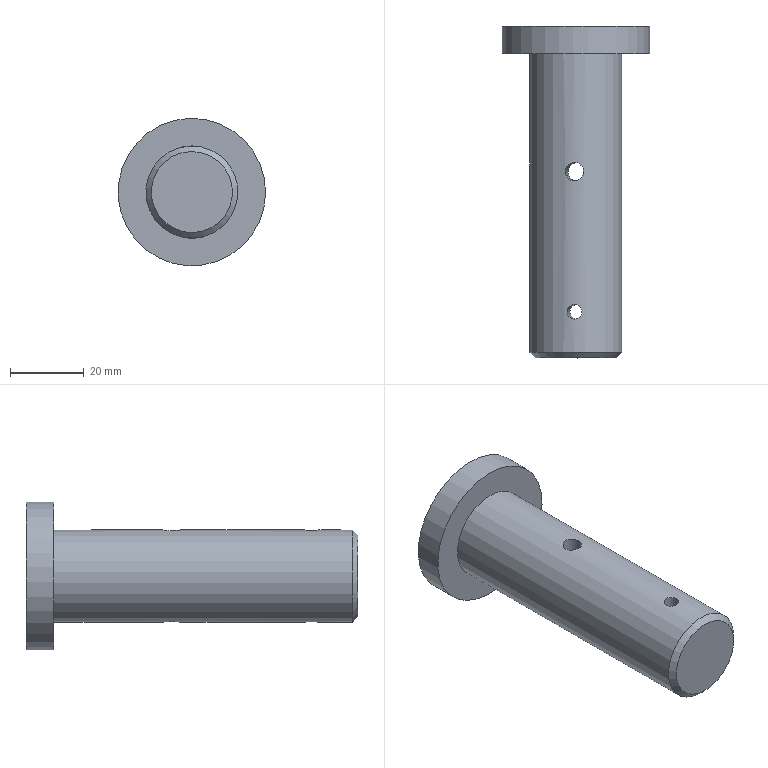Component | NX | 3 | 1 solid | 16 faces | volume 46300 mm3 | cylinder 9 | plane 4 | cone 3 | commonest cylinder face diameters 5 x4 25 x1 40 x1 12.1 x1 4 x1 14 x1